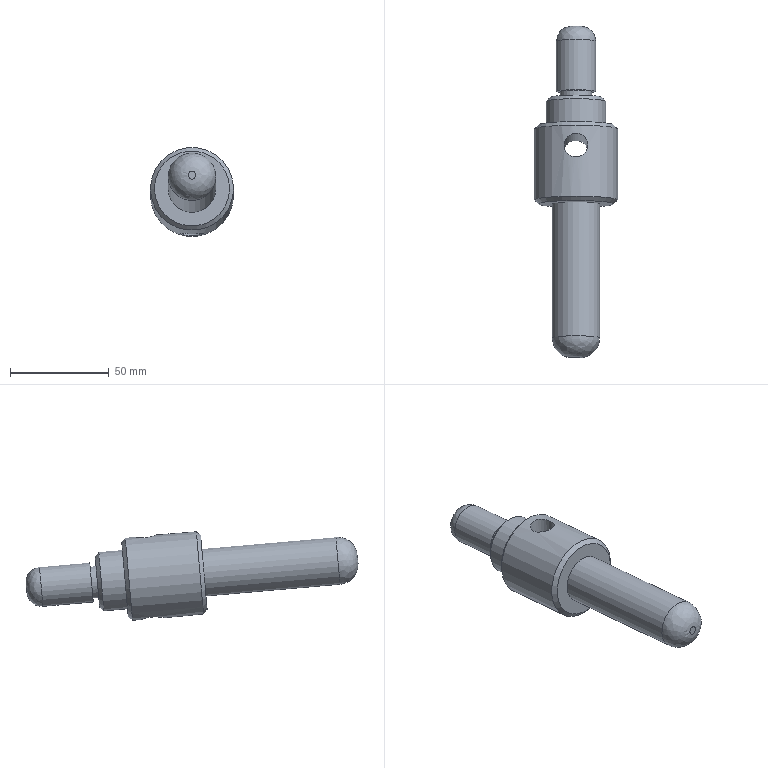Component | NX | LOCATING_PIN | 1 solid | 17 faces | volume 104216 mm3 | cylinder 6 | plane 6 | cone 3 | spline 2 | commonest cylinder face diameters 42 x1 24 x1 30 x1 16 x1 20 x1 12 x1